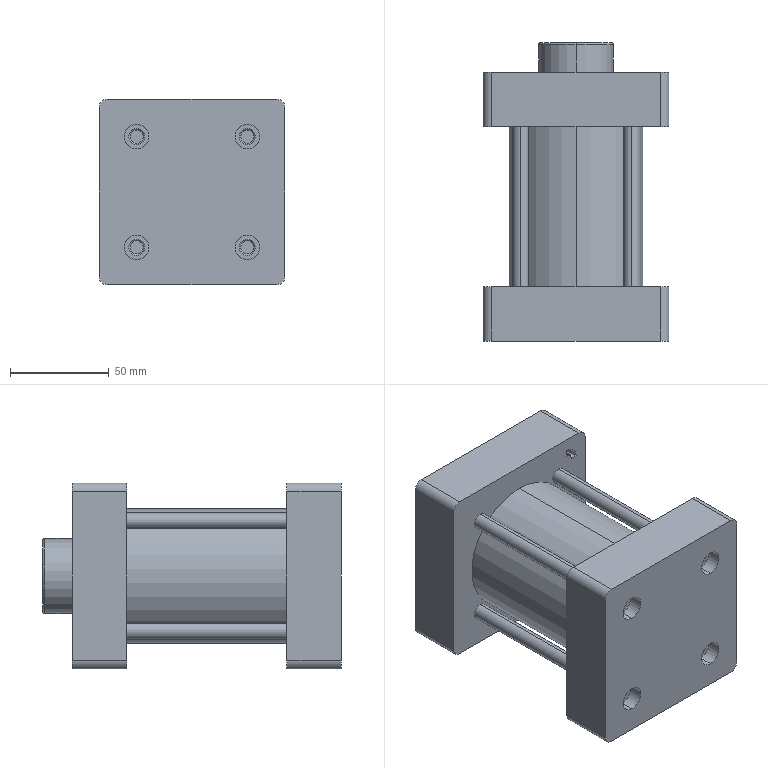Component | SolidWorks | NewCurveBenderSC63x40Cylinder-DoubleWheel-1_NewTypeCurveBenderSC-63x40(0)_c-DoubleWheel-1 | 1 solid | 157 faces | box 94 x 151 x 94 mm | volume 509926 mm3 | cylinder 78 | plane 47 | cone 30 | torus 2 | commonest cylinder face diameters 6.647 x16 12.5 x16 8 x8 8.773 x8 28.4 x4 14.95 x4 5 x4 9.1 x4
build123d program:
from build123d import *

# Parameters (mm, degrees)
BOSS_EXTRUDE1_DEPTH  = 27.5
CUT_REVOLVE1_ANGLE   = 90
SKETCH3_R            = 34
BOSS_EXTRUDE2_DEPTH  = 81
BOSS_EXTRUDE3_START  = -27.5
BOSS_EXTRUDE3_DEPTH  = 27.5
LPATTERN1_COUNT      = 2
LPATTERN1_PITCH      = 56
LPATTERN1_COUNT_DIR2 = 2
LPATTERN1_PITCH_DIR2 = 56
LPATTERN2_COUNT      = 2
LPATTERN2_PITCH      = 56
LPATTERN2_COUNT_DIR2 = 2
LPATTERN2_PITCH_DIR2 = 56
SKETCH9_W            = 81
SKETCH9_H            = 4
LPATTERN3_COUNT      = 2
LPATTERN3_PITCH      = 56
LPATTERN3_COUNT_DIR2 = 2
LPATTERN3_PITCH_DIR2 = 56


with BuildPart() as part:
    # Sketch1 → Boss-Extrude1 (new body)
    with BuildSketch(Plane(origin=(0, 0, 0), x_dir=(0, 0, -1), z_dir=(1, 0, 0))):
        with BuildLine():
            Line((-42.613, -47), (42.613, -47))
            ThreePointArc((42.613, -47), (45.715, -45.715), (47, -42.613))
            Line((47, -42.613), (47, 42.613))
            ThreePointArc((47, 42.613), (45.715, 45.715), (42.613, 47))
            Line((42.613, 47), (-42.613, 47))
            ThreePointArc((-42.613, 47), (-45.715, 45.715), (-47, 42.613))
            Line((-47, 42.613), (-47, -42.613))
            ThreePointArc((-47, -42.613), (-45.715, -45.715), (-42.613, -47))
        make_face()
    extrude(amount=BOSS_EXTRUDE1_DEPTH)

    # Sketch2 → Cut-Revolve1 (revolve, cut)
    with BuildSketch(Plane(origin=(0, 34, 0), x_dir=(1, 0, 0), z_dir=(0, 1, 0))):
        Polygon((0, -37), (0, -40.5), (27.5, -40.5), (27.5, -37), (27, -37.5), (0.5, -37.5), align=None)
    revolve(axis=Axis((0, 34, 34), (-1, 0, 0)), revolution_arc=CUT_REVOLVE1_ANGLE, mode=Mode.SUBTRACT)

    # Sketch3 → Boss-Extrude2 (add)
    with BuildSketch(Plane(origin=(27.5, 0, 0), x_dir=(0, 0, -1), z_dir=(1, 0, 0))):
        Circle(SKETCH3_R)
    extrude(amount=BOSS_EXTRUDE2_DEPTH)

    # Sketch4 → Boss-Extrude3 (add)
    with BuildSketch(Plane(origin=(136, 0, 0), x_dir=(0, 0, -1), z_dir=(1, 0, 0)).offset(BOSS_EXTRUDE3_START)):
        with BuildLine():
            Line((-42.613, -47), (42.613, -47))
            ThreePointArc((42.613, -47), (45.715, -45.715), (47, -42.613))
            Line((47, -42.613), (47, 42.613))
            ThreePointArc((47, 42.613), (45.715, 45.715), (42.613, 47))
            Line((42.613, 47), (-42.613, 47))
            ThreePointArc((-42.613, 47), (-45.715, 45.715), (-47, 42.613))
            Line((-47, 42.613), (-47, -42.613))
            ThreePointArc((-47, -42.613), (-45.715, -45.715), (-42.613, -47))
        make_face()
    extrude(amount=BOSS_EXTRUDE3_DEPTH)

    # Sketch5 → Cut-Revolve2 (revolve, cut)
    with BuildSketch(Plane(origin=(0, -28, 0), x_dir=(1, 0, 0), z_dir=(0, 1, 0))):
        Polygon((18, -28), (18, -31.323), (7.676, -31.323), (7, -32), (7, -34.25), (0, -34.25), (0, -28), align=None)
    cut_revolve2 = revolve(axis=Axis((0, -28, 28), (1, 0, 0)), mode=Mode.SUBTRACT)

    # LPattern1: Cut-Revolve2 2 × 2
    with Locations(*[(0, j * LPATTERN1_PITCH_DIR2, -i * LPATTERN1_PITCH) for i in range(LPATTERN1_COUNT) for j in range(LPATTERN1_COUNT_DIR2) if (i, j) != (0, 0)]):
        add(cut_revolve2, mode=Mode.SUBTRACT)

    # Sketch7 → Cut-Revolve3 (revolve, cut)
    with BuildSketch(Plane(origin=(0, -28, 0), x_dir=(1, 0, 0), z_dir=(0, 1, 0))):
        Polygon((136, -28), (136, -34.25), (129, -34.25), (129, -32), (128.323, -31.323), (118, -31.323), (118, -28), align=None)
    cut_revolve3 = revolve(axis=Axis((118, -28, 28), (1, 0, 0)), mode=Mode.SUBTRACT)

    # LPattern2: Cut-Revolve3 2 × 2
    with Locations(*[(0, j * LPATTERN2_PITCH_DIR2, -i * LPATTERN2_PITCH) for i in range(LPATTERN2_COUNT) for j in range(LPATTERN2_COUNT_DIR2) if (i, j) != (0, 0)]):
        add(cut_revolve3, mode=Mode.SUBTRACT)

    # Sketch9 → Revolve1 (revolve)
    with BuildSketch(Plane(origin=(0, -28, 0), x_dir=(1, 0, 0), z_dir=(0, 1, 0)), mode=Mode.PRIVATE) as revolve1_sk:
        with Locations((68, -26)):
            Rectangle(SKETCH9_W, SKETCH9_H)
    revolve1 = revolve(revolve1_sk.sketch.rotate(Axis((108.5, -28, 28), (-1, 0, 0)), 180), axis=Axis((108.5, -28, 28), (-1, 0, 0)))

    # LPattern3: Revolve1 2 × 2
    with Locations(*[(0, j * LPATTERN3_PITCH_DIR2, -i * LPATTERN3_PITCH) for i in range(LPATTERN3_COUNT) for j in range(LPATTERN3_COUNT_DIR2) if (i, j) != (0, 0)]):
        add(revolve1)

    # Sketch11 → Cut-Revolve4 (revolve, cut)
    with BuildSketch(Plane(origin=(15, 0, 0), x_dir=(0, 0, -1), z_dir=(1, 0, 0)), mode=Mode.PRIVATE) as cut_revolve4_sk:
        Polygon((-37.5, 9.5), (-37.5, 17.831), (-36.644, 16.975), (-17.506, 16.975), (-17.506, 9.5), align=None)
    revolve(cut_revolve4_sk.sketch.rotate(Axis((15, 9.5, 17.506), (0, 0, 1)), 270), axis=Axis((15, 9.5, 17.506), (0, 0, 1)), mode=Mode.SUBTRACT)

    # Sketch12 → Cut-Revolve5 (revolve, cut)
    with BuildSketch(Plane(origin=(121, 0, 0), x_dir=(0, 0, -1), z_dir=(1, 0, 0)), mode=Mode.PRIVATE) as cut_revolve5_sk:
        Polygon((-37.5, 9.5), (-37.5, 17.831), (-36.644, 16.975), (-17.506, 16.975), (-17.506, 9.5), align=None)
    revolve(cut_revolve5_sk.sketch.rotate(Axis((121, 9.5, 17.506), (0, 0, 1)), 270), axis=Axis((121, 9.5, 17.506), (0, 0, 1)), mode=Mode.SUBTRACT)

    # Sketch13 → Cut-Revolve6 (revolve, cut)
    with BuildSketch(Plane(origin=(19, 0, 0), x_dir=(0, 0, -1), z_dir=(1, 0, 0)), mode=Mode.PRIVATE) as cut_revolve6_sk:
        Polygon((-37.5, -8.5), (-37.5, -2.95), (-37, -3.45), (-34, -3.45), (-34, -3.95), (-36.5, -3.95), (-37, -4.45), (-37, -6), (-34, -6), (-34, -8.5), align=None)
    revolve(cut_revolve6_sk.sketch.rotate(Axis((19, -8.5, 34), (0, 0, 1)), 90), axis=Axis((19, -8.5, 34), (0, 0, 1)), mode=Mode.SUBTRACT)

    # Sketch14 → Cut-Revolve7 (revolve, cut)
    with BuildSketch(Plane(origin=(117, 0, 0), x_dir=(0, 0, -1), z_dir=(1, 0, 0)), mode=Mode.PRIVATE) as cut_revolve7_sk:
        Polygon((-37.5, -8.5), (-37.5, -2.95), (-37, -3.45), (-34, -3.45), (-34, -3.95), (-36.5, -3.95), (-37, -4.45), (-37, -6), (-34, -6), (-34, -8.5), align=None)
    revolve(cut_revolve7_sk.sketch.rotate(Axis((117, -8.5, 34), (0, 0, 1)), 90), axis=Axis((117, -8.5, 34), (0, 0, 1)), mode=Mode.SUBTRACT)

    # Sketch15 → Revolve2 (revolve)
    with BuildSketch(Plane.XY, mode=Mode.PRIVATE) as revolve2_sk:
        with BuildLine():
            Line((-15, 0), (-15, 18))
            ThreePointArc((-15, 18), (-14.707, 18.707), (-14, 19))
            Line((-14, 19), (0, 19))
            Line((0, 19), (0, 0))
            Line((0, 0), (-15, 0))
        make_face()
    revolve(revolve2_sk.sketch.rotate(Axis((0, 0, 0), (-1, 0, 0)), 270), axis=Axis((0, 0, 0), (-1, 0, 0)))

    # Sketch16 → Cut-Revolve8 (revolve, cut)
    with BuildSketch(Plane.XY, mode=Mode.PRIVATE) as cut_revolve8_sk:
        Polygon((-20, 0), (-20, 10), (-4, 10), (-4, 14.2), (26, 14.2), (26, 31.5), (104, 31.5), (104, 14.2), (134, 14.2), (134, 0), align=None)
    revolve(cut_revolve8_sk.sketch.rotate(Axis((134, 0, 0), (-1, 0, 0)), 270), axis=Axis((134, 0, 0), (-1, 0, 0)), mode=Mode.SUBTRACT)


solid = part.part

# Placed as in the assembly
solid = solid.moved(Location((50, -301, 0), (0, 0, -90)))